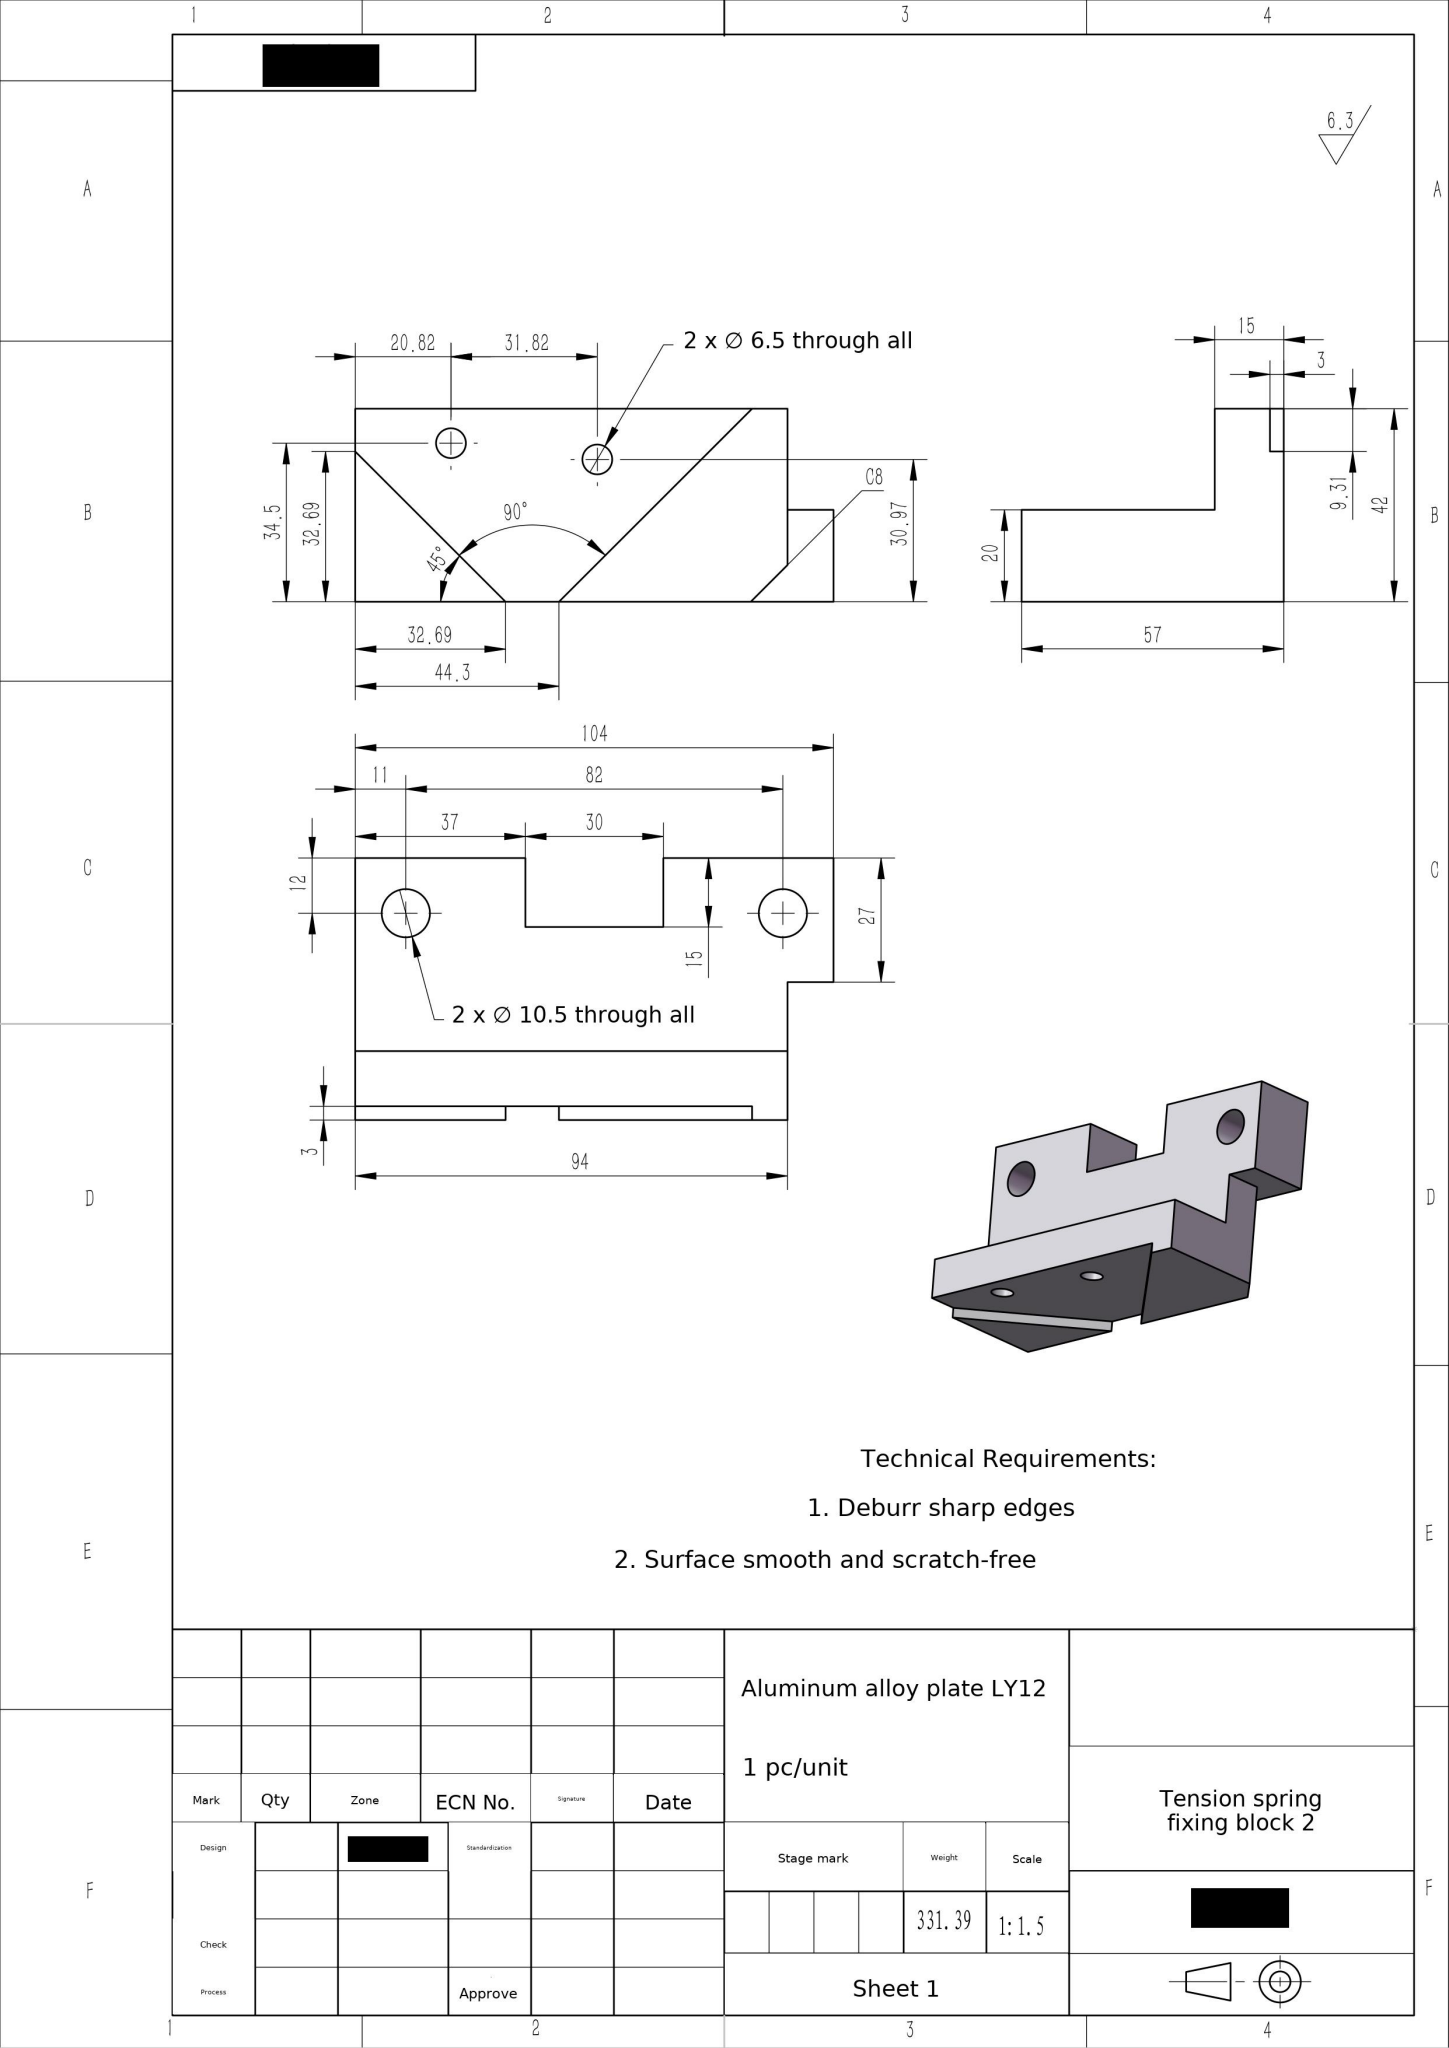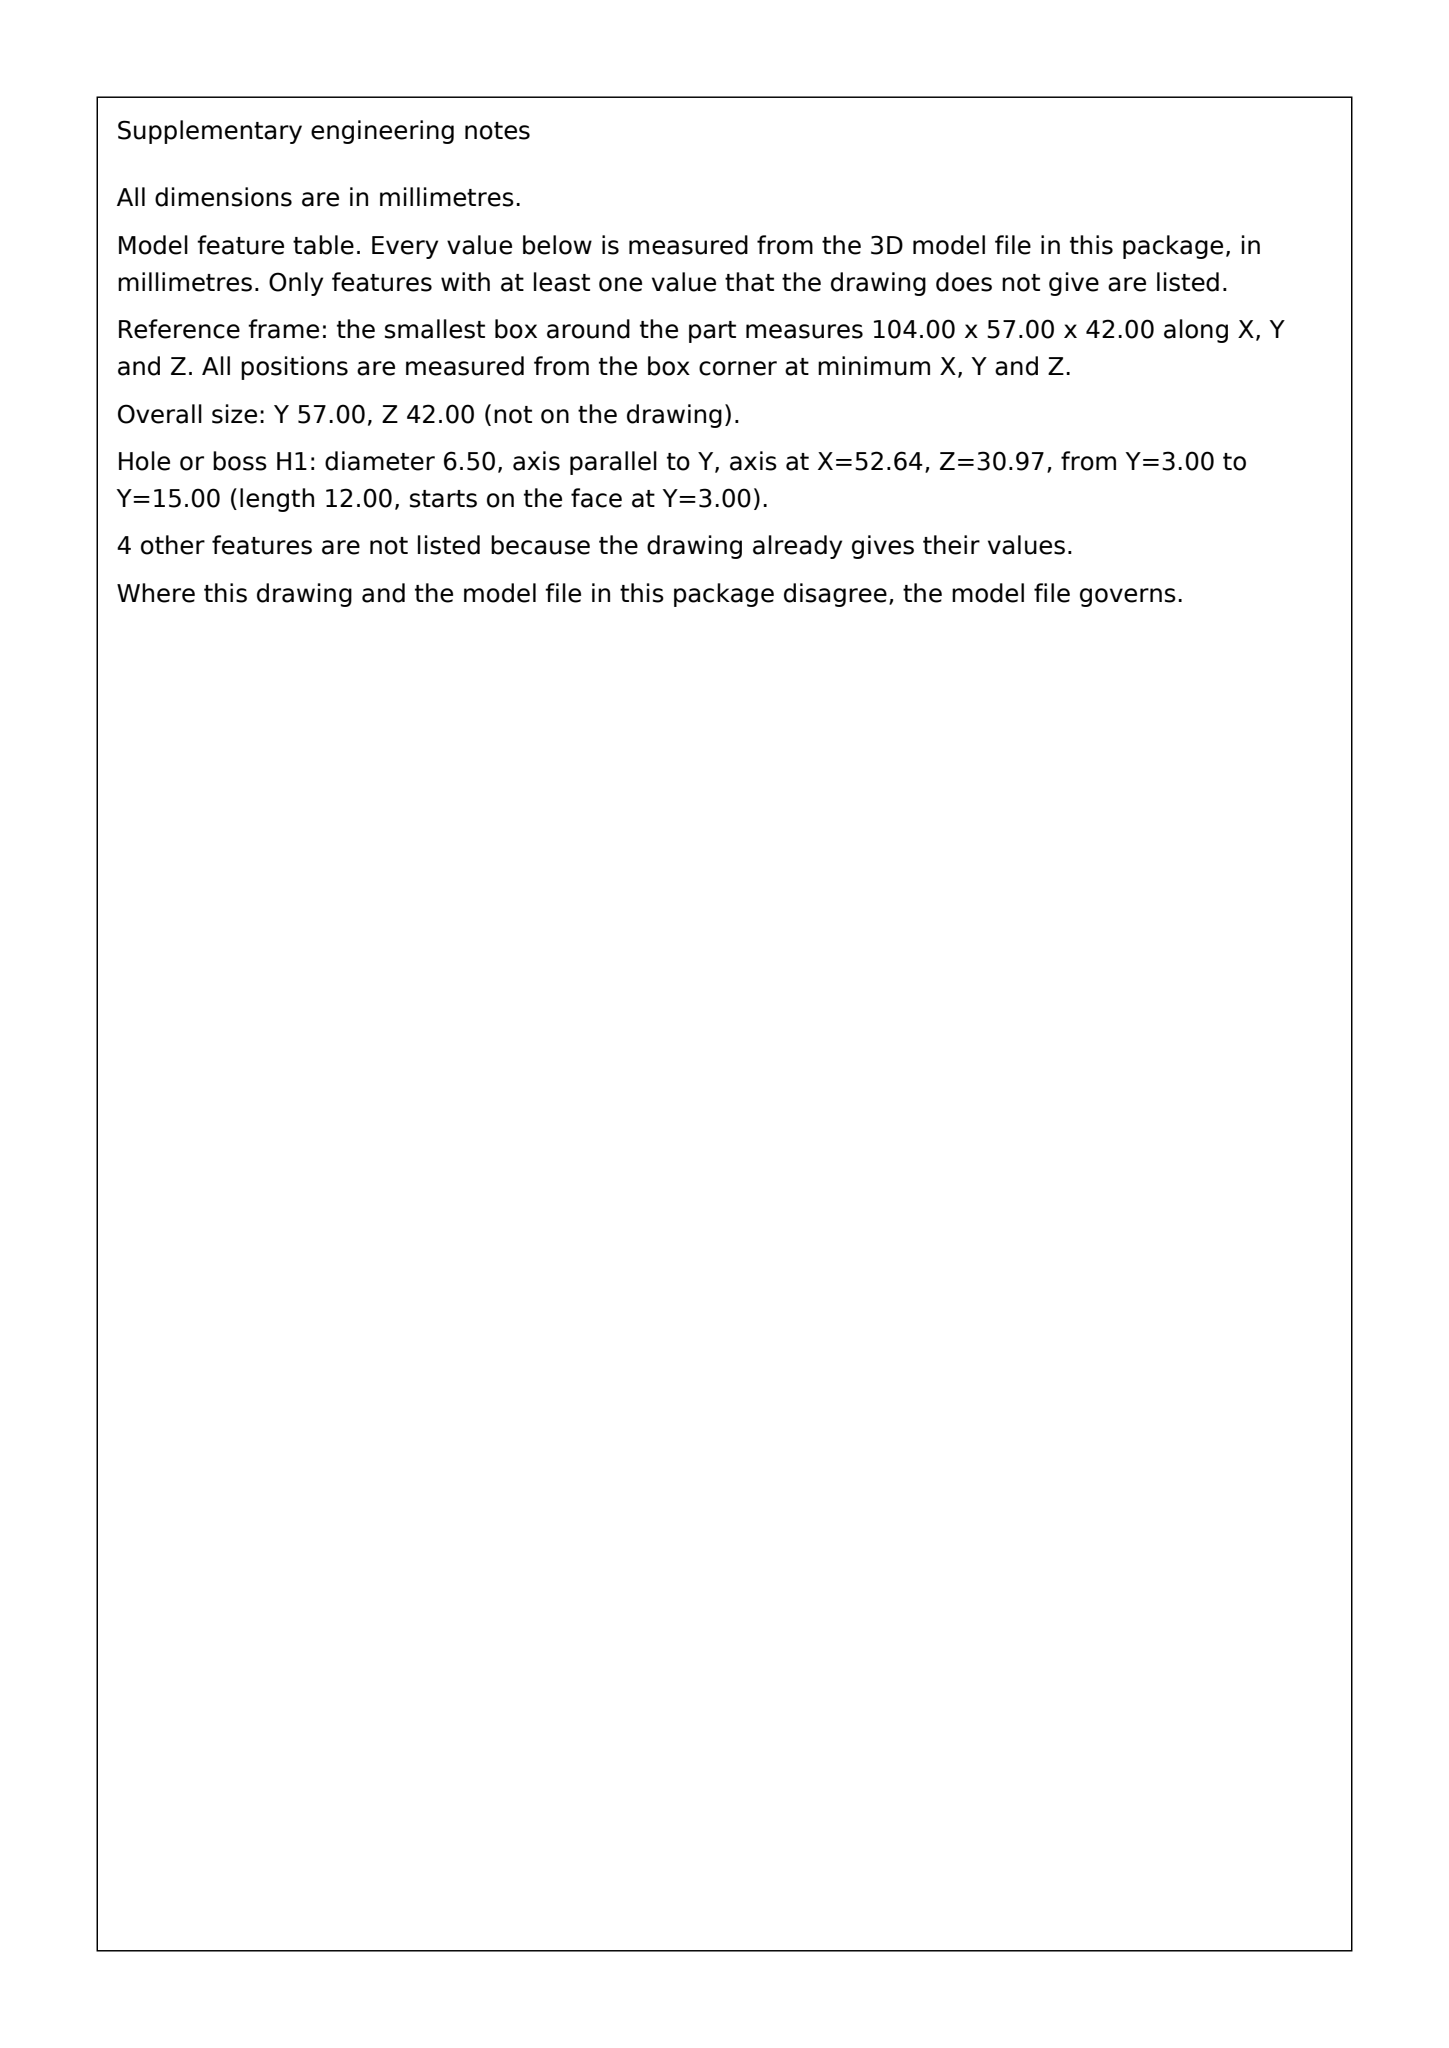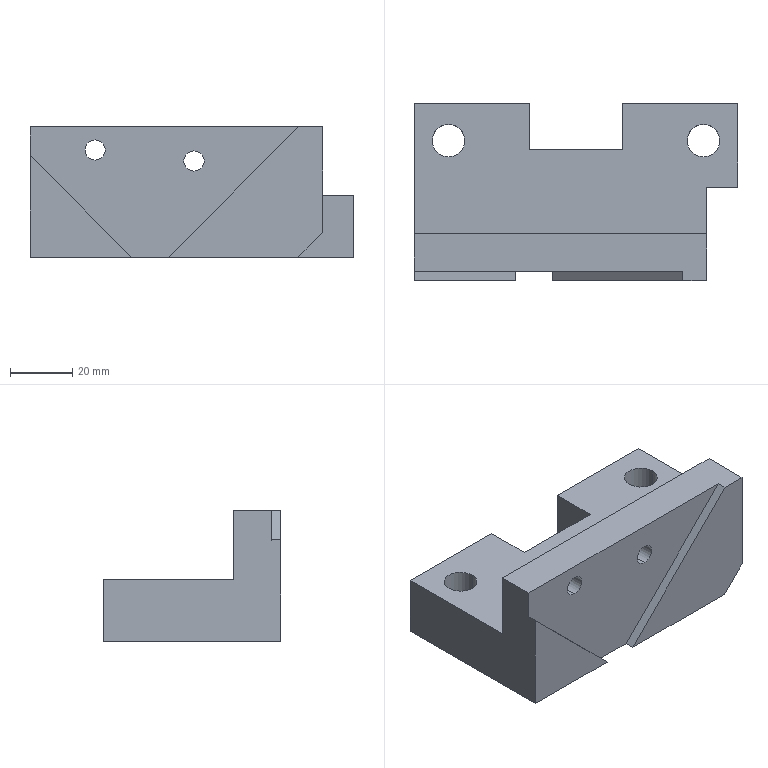Part | SolidWorks | mm | material Aluminum alloy plate LY12 | 1 solid | 27 faces | box 104 x 57 x 42 mm | volume 122736 mm3 | plane 19 | cylinder 8 | commonest cylinder face diameters 6.5 x4 10.5 x4
build123d program:
from build123d import *

# Parameters (mm, degrees)
SKETCH29_W                   = 104
SKETCH29_H                   = 54
BOSS_EXTRUDE1_DEPTH          = 10
SKETCH30_W                   = 30
SKETCH30_H                   = 8
CUT_EXTRUDE7_DEPTH           = 62.911
F_10_5_10_5_DIAMETER_HOLE1_D = 10.5
SKETCH33_W                   = 22
SKETCH33_H                   = 12
BOSS_EXTRUDE2_DEPTH          = 104
BOSS_EXTRUDE3_DEPTH          = 3
F_6_5_6_5_DIAMETER_HOLE1_D   = 6.5
SKETCH37_W                   = 42
SKETCH37_H                   = 30
CUT_EXTRUDE8_DEPTH           = 10
CHAMFER1_SIZE                = 8
MOVE_FACE1_BY                = 7


with BuildPart() as part:
    # Sketch29 → Boss-Extrude1 (new, symmetric)
    with BuildSketch(Plane.XY):
        Rectangle(SKETCH29_W, SKETCH29_H)
    extrude(amount=BOSS_EXTRUDE1_DEPTH, both=True)

    # Sketch30 → Cut-Extrude7 (cut, through all)
    with BuildSketch(Plane.XY.offset(10)):
        with Locations((0, 23)):
            Rectangle(SKETCH30_W, SKETCH30_H)
    extrude(amount=-CUT_EXTRUDE7_DEPTH, mode=Mode.SUBTRACT)

    # 10.5 _10.5_ Diameter Hole1 (through all)
    with Locations(Plane.XY.offset(10)):
        with Locations((-41, 15), (41, 15)):
            Hole(F_10_5_10_5_DIAMETER_HOLE1_D / 2)

    # Sketch33 → Boss-Extrude2 (add, through all)
    with BuildSketch(Plane.ZY.offset(52)):
        with Locations((21, -21)):
            Rectangle(SKETCH33_W, SKETCH33_H)
    extrude(amount=-BOSS_EXTRUDE2_DEPTH)

    # Sketch34 → Boss-Extrude3 (add)
    with BuildSketch(Plane.XZ.offset(27)):
        Polygon((-52, -10), (-19.309, -10), (-52, 22.691), align=None)
        Polygon((-7.703, -10), (34.297, 32), (52, 32), (52, -10), align=None)
    extrude(amount=BOSS_EXTRUDE3_DEPTH)

    # 6.5 _6.5_ Diameter Hole1 (through all)
    with Locations(Plane(origin=(0, -15, 0), x_dir=(1, 0, 0), z_dir=(0, 1, 0))):
        with Locations((-31.183, -24.502), (0.6364, -20.967)):
            Hole(F_6_5_6_5_DIAMETER_HOLE1_D / 2)

    # Sketch37 → Cut-Extrude8 (cut)
    with BuildSketch(Plane(origin=(52, 0, 0), x_dir=(0, 0, -1), z_dir=(1, 0, 0))):
        with Locations((-11, -15)):
            Rectangle(SKETCH37_W, SKETCH37_H)
    extrude(amount=-CUT_EXTRUDE8_DEPTH, mode=Mode.SUBTRACT)

    # Chamfer1
    chamfer1_edges = [part.edges().sort_by_distance(p)[0] for p in [
        (42, -15, -10),
    ]]
    chamfer(chamfer1_edges, length=CHAMFER1_SIZE)

    # Move Face1: a face moved inward by 7.0
    extrude(part.faces().sort_by_distance((0, 19, 0))[0], amount=MOVE_FACE1_BY, dir=(0, -1, 0), mode=Mode.SUBTRACT)


solid = part.part
STEP:
#1=CARTESIAN_POINT('',(-31.183,-27.,21.252));
#2=VERTEX_POINT('',#1);
#3=CARTESIAN_POINT('',(-31.183,-27.,27.752));
#4=VERTEX_POINT('',#3);
#5=CARTESIAN_POINT('',(-31.183,-27.,24.502));
#6=DIRECTION('',(0.,1.,0.));
#7=DIRECTION('',(0.,0.,1.));
#8=AXIS2_PLACEMENT_3D('',#5,#6,#7);
#9=CIRCLE('',#8,3.25);
#10=EDGE_CURVE('',#2,#4,#9,.T.);
#11=ORIENTED_EDGE('',*,*,#10,.F.);
#12=CARTESIAN_POINT('',(-31.183,-15.,21.252));
#13=VERTEX_POINT('',#12);
#14=CARTESIAN_POINT('',(-31.183,-15.,21.252));
#15=DIRECTION('',(0.,1.,0.));
#16=VECTOR('',#15,1000.);
#17=LINE('',#14,#16);
#18=EDGE_CURVE('',#2,#13,#17,.T.);
#19=ORIENTED_EDGE('',*,*,#18,.T.);
#20=CARTESIAN_POINT('',(-31.183,-15.,27.752));
#21=VERTEX_POINT('',#20);
#22=CARTESIAN_POINT('',(-31.183,-15.,24.502));
#23=DIRECTION('',(0.,1.,0.));
#24=DIRECTION('',(0.,0.,1.));
#25=AXIS2_PLACEMENT_3D('',#22,#23,#24);
#26=CIRCLE('',#25,3.25);
#27=EDGE_CURVE('',#13,#21,#26,.T.);
#28=ORIENTED_EDGE('',*,*,#27,.T.);
#29=CARTESIAN_POINT('',(-31.183,-15.,27.752));
#30=DIRECTION('',(0.,1.,0.));
#31=VECTOR('',#30,1000.);
#32=LINE('',#29,#31);
#33=EDGE_CURVE('',#4,#21,#32,.T.);
#34=ORIENTED_EDGE('',*,*,#33,.F.);
#35=EDGE_LOOP('',(#11,#19,#28,#34));
#36=FACE_OUTER_BOUND('',#35,.T.);
#37=CARTESIAN_POINT('',(-31.183,-15.,24.502));
#38=DIRECTION('',(0.,1.,0.));
#39=DIRECTION('',(0.,0.,1.));
#40=AXIS2_PLACEMENT_3D('',#37,#38,#39);
#41=CYLINDRICAL_SURFACE('',#40,3.25);
#42=ADVANCED_FACE('',(#36),#41,.F.);
#43=CARTESIAN_POINT('',(0.6364,-27.,17.717));
#44=VERTEX_POINT('',#43);
#45=CARTESIAN_POINT('',(0.6364,-27.,24.217));
#46=VERTEX_POINT('',#45);
#47=CARTESIAN_POINT('',(0.6364,-27.,20.967));
#48=DIRECTION('',(0.,1.,0.));
#49=DIRECTION('',(0.,0.,1.));
#50=AXIS2_PLACEMENT_3D('',#47,#48,#49);
#51=CIRCLE('',#50,3.25);
#52=EDGE_CURVE('',#44,#46,#51,.T.);
#53=ORIENTED_EDGE('',*,*,#52,.F.);
#54=CARTESIAN_POINT('',(0.6364,-15.,17.717));
#55=VERTEX_POINT('',#54);
#56=CARTESIAN_POINT('',(0.6364,-15.,17.717));
#57=DIRECTION('',(0.,1.,0.));
#58=VECTOR('',#57,1000.);
#59=LINE('',#56,#58);
#60=EDGE_CURVE('',#44,#55,#59,.T.);
#61=ORIENTED_EDGE('',*,*,#60,.T.);
#62=CARTESIAN_POINT('',(0.6364,-15.,24.217));
#63=VERTEX_POINT('',#62);
#64=CARTESIAN_POINT('',(0.6364,-15.,20.967));
#65=DIRECTION('',(0.,1.,0.));
#66=DIRECTION('',(0.,0.,1.));
#67=AXIS2_PLACEMENT_3D('',#64,#65,#66);
#68=CIRCLE('',#67,3.25);
#69=EDGE_CURVE('',#55,#63,#68,.T.);
#70=ORIENTED_EDGE('',*,*,#69,.T.);
#71=CARTESIAN_POINT('',(0.6364,-15.,24.217));
#72=DIRECTION('',(0.,1.,0.));
#73=VECTOR('',#72,1000.);
#74=LINE('',#71,#73);
#75=EDGE_CURVE('',#46,#63,#74,.T.);
#76=ORIENTED_EDGE('',*,*,#75,.F.);
#77=EDGE_LOOP('',(#53,#61,#70,#76));
#78=FACE_OUTER_BOUND('',#77,.T.);
#79=CARTESIAN_POINT('',(0.6364,-15.,20.967));
#80=DIRECTION('',(0.,1.,0.));
#81=DIRECTION('',(0.,0.,1.));
#82=AXIS2_PLACEMENT_3D('',#79,#80,#81);
#83=CYLINDRICAL_SURFACE('',#82,3.25);
#84=ADVANCED_FACE('',(#78),#83,.F.);
#85=CARTESIAN_POINT('',(-46.25,15.,-10.));
#86=VERTEX_POINT('',#85);
#87=CARTESIAN_POINT('',(-35.75,15.,-10.));
#88=VERTEX_POINT('',#87);
#89=CARTESIAN_POINT('',(-41.,15.,-10.));
#90=DIRECTION('',(0.,0.,1.));
#91=DIRECTION('',(1.,0.,0.));
#92=AXIS2_PLACEMENT_3D('',#89,#90,#91);
#93=CIRCLE('',#92,5.25);
#94=EDGE_CURVE('',#86,#88,#93,.T.);
#95=ORIENTED_EDGE('',*,*,#94,.F.);
#96=CARTESIAN_POINT('',(-46.25,15.,10.));
#97=VERTEX_POINT('',#96);
#98=CARTESIAN_POINT('',(-46.25,15.,10.));
#99=DIRECTION('',(0.,0.,1.));
#100=VECTOR('',#99,1000.);
#101=LINE('',#98,#100);
#102=EDGE_CURVE('',#86,#97,#101,.T.);
#103=ORIENTED_EDGE('',*,*,#102,.T.);
#104=CARTESIAN_POINT('',(-35.75,15.,10.));
#105=VERTEX_POINT('',#104);
#106=CARTESIAN_POINT('',(-41.,15.,10.));
#107=DIRECTION('',(0.,0.,1.));
#108=DIRECTION('',(1.,0.,0.));
#109=AXIS2_PLACEMENT_3D('',#106,#107,#108);
#110=CIRCLE('',#109,5.25);
#111=EDGE_CURVE('',#97,#105,#110,.T.);
#112=ORIENTED_EDGE('',*,*,#111,.T.);
#113=CARTESIAN_POINT('',(-35.75,15.,10.));
#114=DIRECTION('',(0.,0.,1.));
#115=VECTOR('',#114,1000.);
#116=LINE('',#113,#115);
#117=EDGE_CURVE('',#88,#105,#116,.T.);
#118=ORIENTED_EDGE('',*,*,#117,.F.);
#119=EDGE_LOOP('',(#95,#103,#112,#118));
#120=FACE_OUTER_BOUND('',#119,.T.);
#121=CARTESIAN_POINT('',(-41.,15.,10.));
#122=DIRECTION('',(0.,0.,1.));
#123=DIRECTION('',(1.,0.,0.));
#124=AXIS2_PLACEMENT_3D('',#121,#122,#123);
#125=CYLINDRICAL_SURFACE('',#124,5.25);
#126=ADVANCED_FACE('',(#120),#125,.F.);
#127=CARTESIAN_POINT('',(35.75,15.,-10.));
#128=VERTEX_POINT('',#127);
#129=CARTESIAN_POINT('',(46.25,15.,-10.));
#130=VERTEX_POINT('',#129);
#131=CARTESIAN_POINT('',(41.,15.,-10.));
#132=DIRECTION('',(0.,0.,1.));
#133=DIRECTION('',(1.,0.,0.));
#134=AXIS2_PLACEMENT_3D('',#131,#132,#133);
#135=CIRCLE('',#134,5.25);
#136=EDGE_CURVE('',#128,#130,#135,.T.);
#137=ORIENTED_EDGE('',*,*,#136,.F.);
#138=CARTESIAN_POINT('',(35.75,15.,10.));
#139=VERTEX_POINT('',#138);
#140=CARTESIAN_POINT('',(35.75,15.,10.));
#141=DIRECTION('',(0.,0.,1.));
#142=VECTOR('',#141,1000.);
#143=LINE('',#140,#142);
#144=EDGE_CURVE('',#128,#139,#143,.T.);
#145=ORIENTED_EDGE('',*,*,#144,.T.);
#146=CARTESIAN_POINT('',(46.25,15.,10.));
#147=VERTEX_POINT('',#146);
#148=CARTESIAN_POINT('',(41.,15.,10.));
#149=DIRECTION('',(0.,0.,1.));
#150=DIRECTION('',(1.,0.,0.));
#151=AXIS2_PLACEMENT_3D('',#148,#149,#150);
#152=CIRCLE('',#151,5.25);
#153=EDGE_CURVE('',#139,#147,#152,.T.);
#154=ORIENTED_EDGE('',*,*,#153,.T.);
#155=CARTESIAN_POINT('',(46.25,15.,10.));
#156=DIRECTION('',(0.,0.,1.));
#157=VECTOR('',#156,1000.);
#158=LINE('',#155,#157);
#159=EDGE_CURVE('',#130,#147,#158,.T.);
#160=ORIENTED_EDGE('',*,*,#159,.F.);
#161=EDGE_LOOP('',(#137,#145,#154,#160));
#162=FACE_OUTER_BOUND('',#161,.T.);
#163=CARTESIAN_POINT('',(41.,15.,10.));
#164=DIRECTION('',(0.,0.,1.));
#165=DIRECTION('',(1.,0.,0.));
#166=AXIS2_PLACEMENT_3D('',#163,#164,#165);
#167=CYLINDRICAL_SURFACE('',#166,5.25);
#168=ADVANCED_FACE('',(#162),#167,.F.);
#169=CARTESIAN_POINT('',(-31.183,-15.,24.502));
#170=DIRECTION('',(0.,1.,0.));
#171=DIRECTION('',(0.,0.,1.));
#172=AXIS2_PLACEMENT_3D('',#169,#170,#171);
#173=CIRCLE('',#172,3.25);
#174=EDGE_CURVE('',#21,#13,#173,.T.);
#175=ORIENTED_EDGE('',*,*,#174,.F.);
#176=ORIENTED_EDGE('',*,*,#27,.F.);
#177=EDGE_LOOP('',(#175,#176));
#178=FACE_BOUND('',#177,.T.);
#179=CARTESIAN_POINT('',(0.6364,-15.,20.967));
#180=DIRECTION('',(0.,1.,0.));
#181=DIRECTION('',(0.,0.,1.));
#182=AXIS2_PLACEMENT_3D('',#179,#180,#181);
#183=CIRCLE('',#182,3.25);
#184=EDGE_CURVE('',#63,#55,#183,.T.);
#185=ORIENTED_EDGE('',*,*,#184,.F.);
#186=ORIENTED_EDGE('',*,*,#69,.F.);
#187=EDGE_LOOP('',(#185,#186));
#188=FACE_BOUND('',#187,.T.);
#189=CARTESIAN_POINT('',(42.,-15.,32.));
#190=VERTEX_POINT('',#189);
#191=CARTESIAN_POINT('',(-52.,-15.,32.));
#192=VERTEX_POINT('',#191);
#193=CARTESIAN_POINT('',(52.,-15.,32.));
#194=DIRECTION('',(-1.,-0.,0.));
#195=VECTOR('',#194,1000.);
#196=LINE('',#193,#195);
#197=EDGE_CURVE('',#190,#192,#196,.T.);
#198=ORIENTED_EDGE('',*,*,#197,.F.);
#199=CARTESIAN_POINT('',(42.,-15.,10.));
#200=VERTEX_POINT('',#199);
#201=CARTESIAN_POINT('',(42.,-15.,10.));
#202=DIRECTION('',(0.,0.,-1.));
#203=VECTOR('',#202,1000.);
#204=LINE('',#201,#203);
#205=EDGE_CURVE('',#190,#200,#204,.T.);
#206=ORIENTED_EDGE('',*,*,#205,.T.);
#207=CARTESIAN_POINT('',(-52.,-15.,10.));
#208=VERTEX_POINT('',#207);
#209=CARTESIAN_POINT('',(52.,-15.,10.));
#210=DIRECTION('',(-1.,-0.,0.));
#211=VECTOR('',#210,1000.);
#212=LINE('',#209,#211);
#213=EDGE_CURVE('',#200,#208,#212,.T.);
#214=ORIENTED_EDGE('',*,*,#213,.T.);
#215=CARTESIAN_POINT('',(-52.,-15.,10.));
#216=DIRECTION('',(0.,0.,-1.));
#217=VECTOR('',#216,1000.);
#218=LINE('',#215,#217);
#219=EDGE_CURVE('',#192,#208,#218,.T.);
#220=ORIENTED_EDGE('',*,*,#219,.F.);
#221=EDGE_LOOP('',(#198,#206,#214,#220));
#222=FACE_OUTER_BOUND('',#221,.T.);
#223=CARTESIAN_POINT('',(52.,-15.,10.));
#224=DIRECTION('',(-0.,1.,0.));
#225=DIRECTION('',(-1.,-0.,0.));
#226=AXIS2_PLACEMENT_3D('',#223,#224,#225);
#227=PLANE('',#226);
#228=ADVANCED_FACE('',(#178,#188,#222),#227,.T.);
#229=CARTESIAN_POINT('',(42.,-30.,32.));
#230=VERTEX_POINT('',#229);
#231=CARTESIAN_POINT('',(34.297,-30.,32.));
#232=VERTEX_POINT('',#231);
#233=CARTESIAN_POINT('',(34.297,-30.,32.));
#234=DIRECTION('',(-1.,0.,0.));
#235=VECTOR('',#234,1000.);
#236=LINE('',#233,#235);
#237=EDGE_CURVE('',#230,#232,#236,.T.);
#238=ORIENTED_EDGE('',*,*,#237,.F.);
#239=CARTESIAN_POINT('',(42.,-30.,32.));
#240=DIRECTION('',(0.,-1.,0.));
#241=VECTOR('',#240,1000.);
#242=LINE('',#239,#241);
#243=EDGE_CURVE('',#190,#230,#242,.T.);
#244=ORIENTED_EDGE('',*,*,#243,.F.);
#245=ORIENTED_EDGE('',*,*,#197,.T.);
#246=CARTESIAN_POINT('',(-52.,-27.,32.));
#247=VERTEX_POINT('',#246);
#248=CARTESIAN_POINT('',(-52.,-27.,32.));
#249=DIRECTION('',(0.,1.,0.));
#250=VECTOR('',#249,1000.);
#251=LINE('',#248,#250);
#252=EDGE_CURVE('',#247,#192,#251,.T.);
#253=ORIENTED_EDGE('',*,*,#252,.F.);
#254=CARTESIAN_POINT('',(34.297,-27.,32.));
#255=VERTEX_POINT('',#254);
#256=CARTESIAN_POINT('',(52.,-27.,32.));
#257=DIRECTION('',(-1.,-0.,0.));
#258=VECTOR('',#257,1000.);
#259=LINE('',#256,#258);
#260=EDGE_CURVE('',#255,#247,#259,.T.);
#261=ORIENTED_EDGE('',*,*,#260,.F.);
#262=CARTESIAN_POINT('',(34.297,-30.,32.));
#263=DIRECTION('',(0.,1.,0.));
#264=VECTOR('',#263,1000.);
#265=LINE('',#262,#264);
#266=EDGE_CURVE('',#232,#255,#265,.T.);
#267=ORIENTED_EDGE('',*,*,#266,.F.);
#268=EDGE_LOOP('',(#238,#244,#245,#253,#261,#267));
#269=FACE_OUTER_BOUND('',#268,.T.);
#270=CARTESIAN_POINT('',(52.,-27.,32.));
#271=DIRECTION('',(0.,0.,1.));
#272=DIRECTION('',(1.,0.,0.));
#273=AXIS2_PLACEMENT_3D('',#270,#271,#272);
#274=PLANE('',#273);
#275=ADVANCED_FACE('',(#269),#274,.T.);
#276=CARTESIAN_POINT('',(-7.703,-30.,-10.));
#277=VERTEX_POINT('',#276);
#278=CARTESIAN_POINT('',(34.,-30.,-10.));
#279=VERTEX_POINT('',#278);
#280=CARTESIAN_POINT('',(52.,-30.,-10.));
#281=DIRECTION('',(1.,0.,0.));
#282=VECTOR('',#281,1000.);
#283=LINE('',#280,#282);
#284=EDGE_CURVE('',#277,#279,#283,.T.);
#285=ORIENTED_EDGE('',*,*,#284,.T.);
#286=CARTESIAN_POINT('',(42.,-30.,-2.));
#287=VERTEX_POINT('',#286);
#288=CARTESIAN_POINT('',(22.,-30.,-22.));
#289=DIRECTION('',(0.7071,0.,0.7071));
#290=VECTOR('',#289,1000.);
#291=LINE('',#288,#290);
#292=EDGE_CURVE('',#279,#287,#291,.T.);
#293=ORIENTED_EDGE('',*,*,#292,.T.);
#294=CARTESIAN_POINT('',(42.,-30.,-10.));
#295=DIRECTION('',(0.,0.,-1.));
#296=VECTOR('',#295,1000.);
#297=LINE('',#294,#296);
#298=EDGE_CURVE('',#230,#287,#297,.T.);
#299=ORIENTED_EDGE('',*,*,#298,.F.);
#300=ORIENTED_EDGE('',*,*,#237,.T.);
#301=CARTESIAN_POINT('',(-7.703,-30.,-10.));
#302=DIRECTION('',(-0.7071,0.,-0.7071));
#303=VECTOR('',#302,1000.);
#304=LINE('',#301,#303);
#305=EDGE_CURVE('',#232,#277,#304,.T.);
#306=ORIENTED_EDGE('',*,*,#305,.T.);
#307=EDGE_LOOP('',(#285,#293,#299,#300,#306));
#308=FACE_OUTER_BOUND('',#307,.T.);
#309=CARTESIAN_POINT('',(0.,-30.,0.));
#310=DIRECTION('',(0.,-1.,0.));
#311=DIRECTION('',(0.,0.,-1.));
#312=AXIS2_PLACEMENT_3D('',#309,#310,#311);
#313=PLANE('',#312);
#314=ADVANCED_FACE('',(#308),#313,.T.);
#315=CARTESIAN_POINT('',(-31.183,-27.,24.502));
#316=DIRECTION('',(0.,1.,0.));
#317=DIRECTION('',(0.,0.,1.));
#318=AXIS2_PLACEMENT_3D('',#315,#316,#317);
#319=CIRCLE('',#318,3.25);
#320=EDGE_CURVE('',#4,#2,#319,.T.);
#321=ORIENTED_EDGE('',*,*,#320,.T.);
#322=ORIENTED_EDGE('',*,*,#10,.T.);
#323=EDGE_LOOP('',(#321,#322));
#324=FACE_BOUND('',#323,.T.);
#325=CARTESIAN_POINT('',(0.6364,-27.,20.967));
#326=DIRECTION('',(0.,1.,0.));
#327=DIRECTION('',(0.,0.,1.));
#328=AXIS2_PLACEMENT_3D('',#325,#326,#327);
#329=CIRCLE('',#328,3.25);
#330=EDGE_CURVE('',#46,#44,#329,.T.);
#331=ORIENTED_EDGE('',*,*,#330,.T.);
#332=ORIENTED_EDGE('',*,*,#52,.T.);
#333=EDGE_LOOP('',(#331,#332));
#334=FACE_BOUND('',#333,.T.);
#335=CARTESIAN_POINT('',(-7.703,-27.,-10.));
#336=VERTEX_POINT('',#335);
#337=CARTESIAN_POINT('',(-7.703,-27.,-10.));
#338=DIRECTION('',(-0.7071,0.,-0.7071));
#339=VECTOR('',#338,1000.);
#340=LINE('',#337,#339);
#341=EDGE_CURVE('',#255,#336,#340,.T.);
#342=ORIENTED_EDGE('',*,*,#341,.F.);
#343=ORIENTED_EDGE('',*,*,#260,.T.);
#344=CARTESIAN_POINT('',(-52.,-27.,22.691));
#345=VERTEX_POINT('',#344);
#346=CARTESIAN_POINT('',(-52.,-27.,10.));
#347=DIRECTION('',(0.,0.,-1.));
#348=VECTOR('',#347,1000.);
#349=LINE('',#346,#348);
#350=EDGE_CURVE('',#247,#345,#349,.T.);
#351=ORIENTED_EDGE('',*,*,#350,.T.);
#352=CARTESIAN_POINT('',(-19.309,-27.,-10.));
#353=VERTEX_POINT('',#352);
#354=CARTESIAN_POINT('',(-19.309,-27.,-10.));
#355=DIRECTION('',(-0.7071,0.,0.7071));
#356=VECTOR('',#355,1000.);
#357=LINE('',#354,#356);
#358=EDGE_CURVE('',#353,#345,#357,.T.);
#359=ORIENTED_EDGE('',*,*,#358,.F.);
#360=CARTESIAN_POINT('',(-52.,-27.,-10.));
#361=DIRECTION('',(1.,0.,0.));
#362=VECTOR('',#361,1000.);
#363=LINE('',#360,#362);
#364=EDGE_CURVE('',#353,#336,#363,.T.);
#365=ORIENTED_EDGE('',*,*,#364,.T.);
#366=EDGE_LOOP('',(#342,#343,#351,#359,#365));
#367=FACE_OUTER_BOUND('',#366,.T.);
#368=CARTESIAN_POINT('',(-52.,-27.,10.));
#369=DIRECTION('',(0.,1.,0.));
#370=DIRECTION('',(0.,0.,1.));
#371=AXIS2_PLACEMENT_3D('',#368,#369,#370);
#372=PLANE('',#371);
#373=ADVANCED_FACE('',(#324,#334,#367),#372,.F.);
#374=CARTESIAN_POINT('',(-15.,27.,10.));
#375=VERTEX_POINT('',#374);
#376=CARTESIAN_POINT('',(-52.,27.,10.));
#377=VERTEX_POINT('',#376);
#378=CARTESIAN_POINT('',(-52.,27.,10.));
#379=DIRECTION('',(-1.,0.,0.));
#380=VECTOR('',#379,1000.);
#381=LINE('',#378,#380);
#382=EDGE_CURVE('',#375,#377,#381,.T.);
#383=ORIENTED_EDGE('',*,*,#382,.F.);
#384=CARTESIAN_POINT('',(-15.,27.,-10.));
#385=VERTEX_POINT('',#384);
#386=CARTESIAN_POINT('',(-15.,27.,-10.));
#387=DIRECTION('',(0.,0.,1.));
#388=VECTOR('',#387,1000.);
#389=LINE('',#386,#388);
#390=EDGE_CURVE('',#385,#375,#389,.T.);
#391=ORIENTED_EDGE('',*,*,#390,.F.);
#392=CARTESIAN_POINT('',(-52.,27.,-10.));
#393=VERTEX_POINT('',#392);
#394=CARTESIAN_POINT('',(-52.,27.,-10.));
#395=DIRECTION('',(-1.,0.,0.));
#396=VECTOR('',#395,1000.);
#397=LINE('',#394,#396);
#398=EDGE_CURVE('',#385,#393,#397,.T.);
#399=ORIENTED_EDGE('',*,*,#398,.T.);
#400=CARTESIAN_POINT('',(-52.,27.,10.));
#401=DIRECTION('',(0.,0.,-1.));
#402=VECTOR('',#401,1000.);
#403=LINE('',#400,#402);
#404=EDGE_CURVE('',#377,#393,#403,.T.);
#405=ORIENTED_EDGE('',*,*,#404,.F.);
#406=EDGE_LOOP('',(#383,#391,#399,#405));
#407=FACE_OUTER_BOUND('',#406,.T.);
#408=CARTESIAN_POINT('',(-52.,27.,10.));
#409=DIRECTION('',(0.,-1.,0.));
#410=DIRECTION('',(0.,0.,-1.));
#411=AXIS2_PLACEMENT_3D('',#408,#409,#410);
#412=PLANE('',#411);
#413=ADVANCED_FACE('',(#407),#412,.F.);
#414=CARTESIAN_POINT('',(52.,-0.,10.));
#415=VERTEX_POINT('',#414);
#416=CARTESIAN_POINT('',(52.,27.,10.));
#417=VERTEX_POINT('',#416);
#418=CARTESIAN_POINT('',(52.,27.,10.));
#419=DIRECTION('',(0.,1.,0.));
#420=VECTOR('',#419,1000.);
#421=LINE('',#418,#420);
#422=EDGE_CURVE('',#415,#417,#421,.T.);
#423=ORIENTED_EDGE('',*,*,#422,.F.);
#424=CARTESIAN_POINT('',(52.,-0.,-10.));
#425=VERTEX_POINT('',#424);
#426=CARTESIAN_POINT('',(52.,-0.,-10.));
#427=DIRECTION('',(0.,-0.,1.));
#428=VECTOR('',#427,1000.);
#429=LINE('',#426,#428);
#430=EDGE_CURVE('',#425,#415,#429,.T.);
#431=ORIENTED_EDGE('',*,*,#430,.F.);
#432=CARTESIAN_POINT('',(52.,27.,-10.));
#433=VERTEX_POINT('',#432);
#434=CARTESIAN_POINT('',(52.,27.,-10.));
#435=DIRECTION('',(0.,1.,0.));
#436=VECTOR('',#435,1000.);
#437=LINE('',#434,#436);
#438=EDGE_CURVE('',#425,#433,#437,.T.);
#439=ORIENTED_EDGE('',*,*,#438,.T.);
#440=CARTESIAN_POINT('',(52.,27.,10.));
#441=DIRECTION('',(0.,0.,-1.));
#442=VECTOR('',#441,1000.);
#443=LINE('',#440,#442);
#444=EDGE_CURVE('',#417,#433,#443,.T.);
#445=ORIENTED_EDGE('',*,*,#444,.F.);
#446=EDGE_LOOP('',(#423,#431,#439,#445));
#447=FACE_OUTER_BOUND('',#446,.T.);
#448=CARTESIAN_POINT('',(52.,27.,10.));
#449=DIRECTION('',(-1.,0.,0.));
#450=DIRECTION('',(0.,0.,1.));
#451=AXIS2_PLACEMENT_3D('',#448,#449,#450);
#452=PLANE('',#451);
#453=ADVANCED_FACE('',(#447),#452,.F.);
#454=CARTESIAN_POINT('',(15.,27.,-10.));
#455=VERTEX_POINT('',#454);
#456=CARTESIAN_POINT('',(-52.,27.,-10.));
#457=DIRECTION('',(-1.,0.,0.));
#458=VECTOR('',#457,1000.);
#459=LINE('',#456,#458);
#460=EDGE_CURVE('',#433,#455,#459,.T.);
#461=ORIENTED_EDGE('',*,*,#460,.T.);
#462=CARTESIAN_POINT('',(15.,27.,10.));
#463=VERTEX_POINT('',#462);
#464=CARTESIAN_POINT('',(15.,27.,-10.));
#465=DIRECTION('',(0.,0.,1.));
#466=VECTOR('',#465,1000.);
#467=LINE('',#464,#466);
#468=EDGE_CURVE('',#455,#463,#467,.T.);
#469=ORIENTED_EDGE('',*,*,#468,.T.);
#470=CARTESIAN_POINT('',(-52.,27.,10.));
#471=DIRECTION('',(-1.,0.,0.));
#472=VECTOR('',#471,1000.);
#473=LINE('',#470,#472);
#474=EDGE_CURVE('',#417,#463,#473,.T.);
#475=ORIENTED_EDGE('',*,*,#474,.F.);
#476=ORIENTED_EDGE('',*,*,#444,.T.);
#477=EDGE_LOOP('',(#461,#469,#475,#476));
#478=FACE_OUTER_BOUND('',#477,.T.);
#479=CARTESIAN_POINT('',(-52.,27.,10.));
#480=DIRECTION('',(0.,-1.,0.));
#481=DIRECTION('',(0.,0.,-1.));
#482=AXIS2_PLACEMENT_3D('',#479,#480,#481);
#483=PLANE('',#482);
#484=ADVANCED_FACE('',(#478),#483,.F.);
#485=CARTESIAN_POINT('',(-52.,-30.,-10.));
#486=VERTEX_POINT('',#485);
#487=CARTESIAN_POINT('',(-52.,27.,-10.));
#488=DIRECTION('',(0.,-1.,0.));
#489=VECTOR('',#488,1000.);
#490=LINE('',#487,#489);
#491=EDGE_CURVE('',#393,#486,#490,.T.);
#492=ORIENTED_EDGE('',*,*,#491,.T.);
#493=CARTESIAN_POINT('',(-52.,-30.,22.691));
#494=VERTEX_POINT('',#493);
#495=CARTESIAN_POINT('',(-52.,-30.,22.691));
#496=DIRECTION('',(0.,0.,-1.));
#497=VECTOR('',#496,1000.);
#498=LINE('',#495,#497);
#499=EDGE_CURVE('',#494,#486,#498,.T.);
#500=ORIENTED_EDGE('',*,*,#499,.F.);
#501=CARTESIAN_POINT('',(-52.,-30.,22.691));
#502=DIRECTION('',(0.,1.,0.));
#503=VECTOR('',#502,1000.);
#504=LINE('',#501,#503);
#505=EDGE_CURVE('',#494,#345,#504,.T.);
#506=ORIENTED_EDGE('',*,*,#505,.T.);
#507=ORIENTED_EDGE('',*,*,#350,.F.);
#508=ORIENTED_EDGE('',*,*,#252,.T.);
#509=ORIENTED_EDGE('',*,*,#219,.T.);
#510=CARTESIAN_POINT('',(-52.,27.,10.));
#511=DIRECTION('',(0.,-1.,0.));
#512=VECTOR('',#511,1000.);
#513=LINE('',#510,#512);
#514=EDGE_CURVE('',#377,#208,#513,.T.);
#515=ORIENTED_EDGE('',*,*,#514,.F.);
#516=ORIENTED_EDGE('',*,*,#404,.T.);
#517=EDGE_LOOP('',(#492,#500,#506,#507,#508,#509,#515,#516));
#518=FACE_OUTER_BOUND('',#517,.T.);
#519=CARTESIAN_POINT('',(-52.,27.,10.));
#520=DIRECTION('',(1.,0.,0.));
#521=DIRECTION('',(-0.,1.,0.));
#522=AXIS2_PLACEMENT_3D('',#519,#520,#521);
#523=PLANE('',#522);
#524=ADVANCED_FACE('',(#518),#523,.F.);
#525=CARTESIAN_POINT('',(42.,-0.,10.));
#526=VERTEX_POINT('',#525);
#527=CARTESIAN_POINT('',(0.,-0.,10.));
#528=DIRECTION('',(-1.,0.,0.));
#529=VECTOR('',#528,1000.);
#530=LINE('',#527,#529);
#531=EDGE_CURVE('',#415,#526,#530,.T.);
#532=ORIENTED_EDGE('',*,*,#531,.F.);
#533=ORIENTED_EDGE('',*,*,#422,.T.);
#534=ORIENTED_EDGE('',*,*,#474,.T.);
#535=CARTESIAN_POINT('',(15.,12.,10.));
#536=VERTEX_POINT('',#535);
#537=CARTESIAN_POINT('',(15.,27.,10.));
#538=DIRECTION('',(-0.,1.,0.));
#539=VECTOR('',#538,1000.);
#540=LINE('',#537,#539);
#541=EDGE_CURVE('',#536,#463,#540,.T.);
#542=ORIENTED_EDGE('',*,*,#541,.F.);
#543=CARTESIAN_POINT('',(-15.,12.,10.));
#544=VERTEX_POINT('',#543);
#545=CARTESIAN_POINT('',(-15.,12.,10.));
#546=DIRECTION('',(1.,0.,0.));
#547=VECTOR('',#546,1000.);
#548=LINE('',#545,#547);
#549=EDGE_CURVE('',#544,#536,#548,.T.);
#550=ORIENTED_EDGE('',*,*,#549,.F.);
#551=CARTESIAN_POINT('',(-15.,27.,10.));
#552=DIRECTION('',(-0.,-1.,0.));
#553=VECTOR('',#552,1000.);
#554=LINE('',#551,#553);
#555=EDGE_CURVE('',#375,#544,#554,.T.);
#556=ORIENTED_EDGE('',*,*,#555,.F.);
#557=ORIENTED_EDGE('',*,*,#382,.T.);
#558=ORIENTED_EDGE('',*,*,#514,.T.);
#559=ORIENTED_EDGE('',*,*,#213,.F.);
#560=CARTESIAN_POINT('',(42.,0.,10.));
#561=DIRECTION('',(0.,1.,0.));
#562=VECTOR('',#561,1000.);
#563=LINE('',#560,#562);
#564=EDGE_CURVE('',#200,#526,#563,.T.);
#565=ORIENTED_EDGE('',*,*,#564,.T.);
#566=EDGE_LOOP('',(#532,#533,#534,#542,#550,#556,#557,#558,#559,#565));
#567=FACE_OUTER_BOUND('',#566,.T.);
#568=CARTESIAN_POINT('',(-41.,15.,10.));
#569=DIRECTION('',(0.,0.,1.));
#570=DIRECTION('',(1.,0.,0.));
#571=AXIS2_PLACEMENT_3D('',#568,#569,#570);
#572=CIRCLE('',#571,5.25);
#573=EDGE_CURVE('',#105,#97,#572,.T.);
#574=ORIENTED_EDGE('',*,*,#573,.F.);
#575=ORIENTED_EDGE('',*,*,#111,.F.);
#576=EDGE_LOOP('',(#574,#575));
#577=FACE_BOUND('',#576,.T.);
#578=CARTESIAN_POINT('',(41.,15.,10.));
#579=DIRECTION('',(0.,0.,1.));
#580=DIRECTION('',(1.,0.,0.));
#581=AXIS2_PLACEMENT_3D('',#578,#579,#580);
#582=CIRCLE('',#581,5.25);
#583=EDGE_CURVE('',#147,#139,#582,.T.);
#584=ORIENTED_EDGE('',*,*,#583,.F.);
#585=ORIENTED_EDGE('',*,*,#153,.F.);
#586=EDGE_LOOP('',(#584,#585));
#587=FACE_BOUND('',#586,.T.);
#588=CARTESIAN_POINT('',(0.,0.,10.));
#589=DIRECTION('',(0.,0.,1.));
#590=DIRECTION('',(1.,0.,0.));
#591=AXIS2_PLACEMENT_3D('',#588,#589,#590);
#592=PLANE('',#591);
#593=ADVANCED_FACE('',(#567,#577,#587),#592,.T.);
#594=CARTESIAN_POINT('',(-41.,15.,-10.));
#595=DIRECTION('',(0.,0.,1.));
#596=DIRECTION('',(1.,0.,0.));
#597=AXIS2_PLACEMENT_3D('',#594,#595,#596);
#598=CIRCLE('',#597,5.25);
#599=EDGE_CURVE('',#88,#86,#598,.T.);
#600=ORIENTED_EDGE('',*,*,#599,.T.);
#601=ORIENTED_EDGE('',*,*,#94,.T.);
#602=EDGE_LOOP('',(#600,#601));
#603=FACE_BOUND('',#602,.T.);
#604=CARTESIAN_POINT('',(41.,15.,-10.));
#605=DIRECTION('',(0.,0.,1.));
#606=DIRECTION('',(1.,0.,0.));
#607=AXIS2_PLACEMENT_3D('',#604,#605,#606);
#608=CIRCLE('',#607,5.25);
#609=EDGE_CURVE('',#130,#128,#608,.T.);
#610=ORIENTED_EDGE('',*,*,#609,.T.);
#611=ORIENTED_EDGE('',*,*,#136,.T.);
#612=EDGE_LOOP('',(#610,#611));
#613=FACE_BOUND('',#612,.T.);
#614=CARTESIAN_POINT('',(34.,-0.,-10.));
#615=VERTEX_POINT('',#614);
#616=CARTESIAN_POINT('',(42.,-0.,-10.));
#617=DIRECTION('',(1.,0.,0.));
#618=VECTOR('',#617,1000.);
#619=LINE('',#616,#618);
#620=EDGE_CURVE('',#615,#425,#619,.T.);
#621=ORIENTED_EDGE('',*,*,#620,.F.);
#622=CARTESIAN_POINT('',(34.,-30.,-10.));
#623=DIRECTION('',(0.,-1.,0.));
#624=VECTOR('',#623,1000.);
#625=LINE('',#622,#624);
#626=EDGE_CURVE('',#615,#279,#625,.T.);
#627=ORIENTED_EDGE('',*,*,#626,.T.);
#628=ORIENTED_EDGE('',*,*,#284,.F.);
#629=CARTESIAN_POINT('',(-7.703,-30.,-10.));
#630=DIRECTION('',(0.,1.,0.));
#631=VECTOR('',#630,1000.);
#632=LINE('',#629,#631);
#633=EDGE_CURVE('',#277,#336,#632,.T.);
#634=ORIENTED_EDGE('',*,*,#633,.T.);
#635=ORIENTED_EDGE('',*,*,#364,.F.);
#636=CARTESIAN_POINT('',(-19.309,-30.,-10.));
#637=VERTEX_POINT('',#636);
#638=CARTESIAN_POINT('',(-19.309,-30.,-10.));
#639=DIRECTION('',(0.,1.,0.));
#640=VECTOR('',#639,1000.);
#641=LINE('',#638,#640);
#642=EDGE_CURVE('',#637,#353,#641,.T.);
#643=ORIENTED_EDGE('',*,*,#642,.F.);
#644=CARTESIAN_POINT('',(-52.,-30.,-10.));
#645=DIRECTION('',(1.,0.,0.));
#646=VECTOR('',#645,1000.);
#647=LINE('',#644,#646);
#648=EDGE_CURVE('',#486,#637,#647,.T.);
#649=ORIENTED_EDGE('',*,*,#648,.F.);
#650=ORIENTED_EDGE('',*,*,#491,.F.);
#651=ORIENTED_EDGE('',*,*,#398,.F.);
#652=CARTESIAN_POINT('',(-15.,12.,-10.));
#653=VERTEX_POINT('',#652);
#654=CARTESIAN_POINT('',(-15.,27.,-10.));
#655=DIRECTION('',(-0.,-1.,0.));
#656=VECTOR('',#655,1000.);
#657=LINE('',#654,#656);
#658=EDGE_CURVE('',#385,#653,#657,.T.);
#659=ORIENTED_EDGE('',*,*,#658,.T.);
#660=CARTESIAN_POINT('',(15.,12.,-10.));
#661=VERTEX_POINT('',#660);
#662=CARTESIAN_POINT('',(-15.,12.,-10.));
#663=DIRECTION('',(1.,0.,0.));
#664=VECTOR('',#663,1000.);
#665=LINE('',#662,#664);
#666=EDGE_CURVE('',#653,#661,#665,.T.);
#667=ORIENTED_EDGE('',*,*,#666,.T.);
#668=CARTESIAN_POINT('',(15.,27.,-10.));
#669=DIRECTION('',(-0.,1.,0.));
#670=VECTOR('',#669,1000.);
#671=LINE('',#668,#670);
#672=EDGE_CURVE('',#661,#455,#671,.T.);
#673=ORIENTED_EDGE('',*,*,#672,.T.);
#674=ORIENTED_EDGE('',*,*,#460,.F.);
#675=ORIENTED_EDGE('',*,*,#438,.F.);
#676=EDGE_LOOP('',(#621,#627,#628,#634,#635,#643,#649,#650,#651,#659,#667,#673,#674,#675));
#677=FACE_OUTER_BOUND('',#676,.T.);
#678=CARTESIAN_POINT('',(0.,0.,-10.));
#679=DIRECTION('',(0.,0.,1.));
#680=DIRECTION('',(1.,0.,0.));
#681=AXIS2_PLACEMENT_3D('',#678,#679,#680);
#682=PLANE('',#681);
#683=ADVANCED_FACE('',(#603,#613,#677),#682,.F.);
#684=ORIENTED_EDGE('',*,*,#555,.T.);
#685=CARTESIAN_POINT('',(-15.,12.,-10.));
#686=DIRECTION('',(0.,0.,1.));
#687=VECTOR('',#686,1000.);
#688=LINE('',#685,#687);
#689=EDGE_CURVE('',#653,#544,#688,.T.);
#690=ORIENTED_EDGE('',*,*,#689,.F.);
#691=ORIENTED_EDGE('',*,*,#658,.F.);
#692=ORIENTED_EDGE('',*,*,#390,.T.);
#693=EDGE_LOOP('',(#684,#690,#691,#692));
#694=FACE_OUTER_BOUND('',#693,.T.);
#695=CARTESIAN_POINT('',(-15.,27.,-10.));
#696=DIRECTION('',(-1.,0.,0.));
#697=DIRECTION('',(-0.,-1.,0.));
#698=AXIS2_PLACEMENT_3D('',#695,#696,#697);
#699=PLANE('',#698);
#700=ADVANCED_FACE('',(#694),#699,.F.);
#701=ORIENTED_EDGE('',*,*,#541,.T.);
#702=ORIENTED_EDGE('',*,*,#468,.F.);
#703=ORIENTED_EDGE('',*,*,#672,.F.);
#704=CARTESIAN_POINT('',(15.,12.,-10.));
#705=DIRECTION('',(0.,0.,1.));
#706=VECTOR('',#705,1000.);
#707=LINE('',#704,#706);
#708=EDGE_CURVE('',#661,#536,#707,.T.);
#709=ORIENTED_EDGE('',*,*,#708,.T.);
#710=EDGE_LOOP('',(#701,#702,#703,#709));
#711=FACE_OUTER_BOUND('',#710,.T.);
#712=CARTESIAN_POINT('',(15.,27.,-10.));
#713=DIRECTION('',(1.,0.,0.));
#714=DIRECTION('',(-0.,1.,0.));
#715=AXIS2_PLACEMENT_3D('',#712,#713,#714);
#716=PLANE('',#715);
#717=ADVANCED_FACE('',(#711),#716,.F.);
#718=ORIENTED_EDGE('',*,*,#549,.T.);
#719=ORIENTED_EDGE('',*,*,#708,.F.);
#720=ORIENTED_EDGE('',*,*,#666,.F.);
#721=ORIENTED_EDGE('',*,*,#689,.T.);
#722=EDGE_LOOP('',(#718,#719,#720,#721));
#723=FACE_OUTER_BOUND('',#722,.T.);
#724=CARTESIAN_POINT('',(-15.,12.,-10.));
#725=DIRECTION('',(0.,-1.,0.));
#726=DIRECTION('',(0.,0.,-1.));
#727=AXIS2_PLACEMENT_3D('',#724,#725,#726);
#728=PLANE('',#727);
#729=ADVANCED_FACE('',(#723),#728,.F.);
#730=ORIENTED_EDGE('',*,*,#144,.F.);
#731=ORIENTED_EDGE('',*,*,#609,.F.);
#732=ORIENTED_EDGE('',*,*,#159,.T.);
#733=ORIENTED_EDGE('',*,*,#583,.T.);
#734=EDGE_LOOP('',(#730,#731,#732,#733));
#735=FACE_OUTER_BOUND('',#734,.T.);
#736=CARTESIAN_POINT('',(41.,15.,10.));
#737=DIRECTION('',(0.,0.,1.));
#738=DIRECTION('',(1.,0.,0.));
#739=AXIS2_PLACEMENT_3D('',#736,#737,#738);
#740=CYLINDRICAL_SURFACE('',#739,5.25);
#741=ADVANCED_FACE('',(#735),#740,.F.);
#742=ORIENTED_EDGE('',*,*,#102,.F.);
#743=ORIENTED_EDGE('',*,*,#599,.F.);
#744=ORIENTED_EDGE('',*,*,#117,.T.);
#745=ORIENTED_EDGE('',*,*,#573,.T.);
#746=EDGE_LOOP('',(#742,#743,#744,#745));
#747=FACE_OUTER_BOUND('',#746,.T.);
#748=CARTESIAN_POINT('',(-41.,15.,10.));
#749=DIRECTION('',(0.,0.,1.));
#750=DIRECTION('',(1.,0.,0.));
#751=AXIS2_PLACEMENT_3D('',#748,#749,#750);
#752=CYLINDRICAL_SURFACE('',#751,5.25);
#753=ADVANCED_FACE('',(#747),#752,.F.);
#754=ORIENTED_EDGE('',*,*,#358,.T.);
#755=ORIENTED_EDGE('',*,*,#505,.F.);
#756=CARTESIAN_POINT('',(-19.309,-30.,-10.));
#757=DIRECTION('',(-0.7071,0.,0.7071));
#758=VECTOR('',#757,1000.);
#759=LINE('',#756,#758);
#760=EDGE_CURVE('',#637,#494,#759,.T.);
#761=ORIENTED_EDGE('',*,*,#760,.F.);
#762=ORIENTED_EDGE('',*,*,#642,.T.);
#763=EDGE_LOOP('',(#754,#755,#761,#762));
#764=FACE_OUTER_BOUND('',#763,.T.);
#765=CARTESIAN_POINT('',(-19.309,-30.,-10.));
#766=DIRECTION('',(-0.7071,0.,-0.7071));
#767=DIRECTION('',(-0.7071,0.,0.7071));
#768=AXIS2_PLACEMENT_3D('',#765,#766,#767);
#769=PLANE('',#768);
#770=ADVANCED_FACE('',(#764),#769,.F.);
#771=ORIENTED_EDGE('',*,*,#499,.T.);
#772=ORIENTED_EDGE('',*,*,#648,.T.);
#773=ORIENTED_EDGE('',*,*,#760,.T.);
#774=EDGE_LOOP('',(#771,#772,#773));
#775=FACE_OUTER_BOUND('',#774,.T.);
#776=CARTESIAN_POINT('',(0.,-30.,0.));
#777=DIRECTION('',(0.,-1.,0.));
#778=DIRECTION('',(0.,0.,-1.));
#779=AXIS2_PLACEMENT_3D('',#776,#777,#778);
#780=PLANE('',#779);
#781=ADVANCED_FACE('',(#775),#780,.T.);
#782=ORIENTED_EDGE('',*,*,#341,.T.);
#783=ORIENTED_EDGE('',*,*,#633,.F.);
#784=ORIENTED_EDGE('',*,*,#305,.F.);
#785=ORIENTED_EDGE('',*,*,#266,.T.);
#786=EDGE_LOOP('',(#782,#783,#784,#785));
#787=FACE_OUTER_BOUND('',#786,.T.);
#788=CARTESIAN_POINT('',(-7.703,-30.,-10.));
#789=DIRECTION('',(0.7071,0.,-0.7071));
#790=DIRECTION('',(-0.7071,0.,-0.7071));
#791=AXIS2_PLACEMENT_3D('',#788,#789,#790);
#792=PLANE('',#791);
#793=ADVANCED_FACE('',(#787),#792,.F.);
#794=ORIENTED_EDGE('',*,*,#60,.F.);
#795=ORIENTED_EDGE('',*,*,#330,.F.);
#796=ORIENTED_EDGE('',*,*,#75,.T.);
#797=ORIENTED_EDGE('',*,*,#184,.T.);
#798=EDGE_LOOP('',(#794,#795,#796,#797));
#799=FACE_OUTER_BOUND('',#798,.T.);
#800=CARTESIAN_POINT('',(0.6364,-15.,20.967));
#801=DIRECTION('',(0.,1.,0.));
#802=DIRECTION('',(0.,0.,1.));
#803=AXIS2_PLACEMENT_3D('',#800,#801,#802);
#804=CYLINDRICAL_SURFACE('',#803,3.25);
#805=ADVANCED_FACE('',(#799),#804,.F.);
#806=ORIENTED_EDGE('',*,*,#18,.F.);
#807=ORIENTED_EDGE('',*,*,#320,.F.);
#808=ORIENTED_EDGE('',*,*,#33,.T.);
#809=ORIENTED_EDGE('',*,*,#174,.T.);
#810=EDGE_LOOP('',(#806,#807,#808,#809));
#811=FACE_OUTER_BOUND('',#810,.T.);
#812=CARTESIAN_POINT('',(-31.183,-15.,24.502));
#813=DIRECTION('',(0.,1.,0.));
#814=DIRECTION('',(0.,0.,1.));
#815=AXIS2_PLACEMENT_3D('',#812,#813,#814);
#816=CYLINDRICAL_SURFACE('',#815,3.25);
#817=ADVANCED_FACE('',(#811),#816,.F.);
#818=ORIENTED_EDGE('',*,*,#531,.T.);
#819=CARTESIAN_POINT('',(42.,-0.,-2.));
#820=VERTEX_POINT('',#819);
#821=CARTESIAN_POINT('',(42.,-0.,-10.));
#822=DIRECTION('',(0.,-0.,1.));
#823=VECTOR('',#822,1000.);
#824=LINE('',#821,#823);
#825=EDGE_CURVE('',#820,#526,#824,.T.);
#826=ORIENTED_EDGE('',*,*,#825,.F.);
#827=CARTESIAN_POINT('',(38.,-0.,-6.));
#828=DIRECTION('',(-0.7071,0.,-0.7071));
#829=VECTOR('',#828,1000.);
#830=LINE('',#827,#829);
#831=EDGE_CURVE('',#820,#615,#830,.T.);
#832=ORIENTED_EDGE('',*,*,#831,.T.);
#833=ORIENTED_EDGE('',*,*,#620,.T.);
#834=ORIENTED_EDGE('',*,*,#430,.T.);
#835=EDGE_LOOP('',(#818,#826,#832,#833,#834));
#836=FACE_OUTER_BOUND('',#835,.T.);
#837=CARTESIAN_POINT('',(42.,-0.,-10.));
#838=DIRECTION('',(0.,1.,0.));
#839=DIRECTION('',(0.,-0.,1.));
#840=AXIS2_PLACEMENT_3D('',#837,#838,#839);
#841=PLANE('',#840);
#842=ADVANCED_FACE('',(#836),#841,.F.);
#843=ORIENTED_EDGE('',*,*,#298,.T.);
#844=CARTESIAN_POINT('',(42.,-0.,-2.));
#845=DIRECTION('',(0.,1.,0.));
#846=VECTOR('',#845,1000.);
#847=LINE('',#844,#846);
#848=EDGE_CURVE('',#287,#820,#847,.T.);
#849=ORIENTED_EDGE('',*,*,#848,.T.);
#850=ORIENTED_EDGE('',*,*,#825,.T.);
#851=ORIENTED_EDGE('',*,*,#564,.F.);
#852=ORIENTED_EDGE('',*,*,#205,.F.);
#853=ORIENTED_EDGE('',*,*,#243,.T.);
#854=EDGE_LOOP('',(#843,#849,#850,#851,#852,#853));
#855=FACE_OUTER_BOUND('',#854,.T.);
#856=CARTESIAN_POINT('',(42.,0.,0.));
#857=DIRECTION('',(1.,0.,0.));
#858=DIRECTION('',(0.,0.,-1.));
#859=AXIS2_PLACEMENT_3D('',#856,#857,#858);
#860=PLANE('',#859);
#861=ADVANCED_FACE('',(#855),#860,.T.);
#862=ORIENTED_EDGE('',*,*,#292,.F.);
#863=ORIENTED_EDGE('',*,*,#626,.F.);
#864=ORIENTED_EDGE('',*,*,#831,.F.);
#865=ORIENTED_EDGE('',*,*,#848,.F.);
#866=EDGE_LOOP('',(#862,#863,#864,#865));
#867=FACE_OUTER_BOUND('',#866,.T.);
#868=CARTESIAN_POINT('',(42.,0.,-2.));
#869=DIRECTION('',(0.7071,0.,-0.7071));
#870=DIRECTION('',(0.,-1.,0.));
#871=AXIS2_PLACEMENT_3D('',#868,#869,#870);
#872=PLANE('',#871);
#873=ADVANCED_FACE('',(#867),#872,.T.);
#874=CLOSED_SHELL('',(#42,#84,#126,#168,#228,#275,#314,#373,#413,#453,#484,#524,#593,#683,#700,#717,#729,#741,#753,#770,#781,#793,#805,#817,#842,#861,#873));
#875=MANIFOLD_SOLID_BREP('',#874);
#876=CARTESIAN_POINT('',(0.,0.,0.));
#877=DIRECTION('',(0.,0.,1.));
#878=DIRECTION('',(1.,0.,0.));
#879=AXIS2_PLACEMENT_3D('',#876,#877,#878);
#880=(LENGTH_UNIT()NAMED_UNIT(*)SI_UNIT(.MILLI.,.METRE.));
#881=UNCERTAINTY_MEASURE_WITH_UNIT(LENGTH_MEASURE(0.00001),#880,'','');
#882=(NAMED_UNIT(*)PLANE_ANGLE_UNIT()SI_UNIT($,.RADIAN.));
#883=(NAMED_UNIT(*)SI_UNIT($,.STERADIAN.)SOLID_ANGLE_UNIT());
#884=(GEOMETRIC_REPRESENTATION_CONTEXT(3)GLOBAL_UNCERTAINTY_ASSIGNED_CONTEXT((#881))GLOBAL_UNIT_ASSIGNED_CONTEXT((#880,#882,#883))REPRESENTATION_CONTEXT('',''));
#885=ADVANCED_BREP_SHAPE_REPRESENTATION('',(#875,#879),#884);